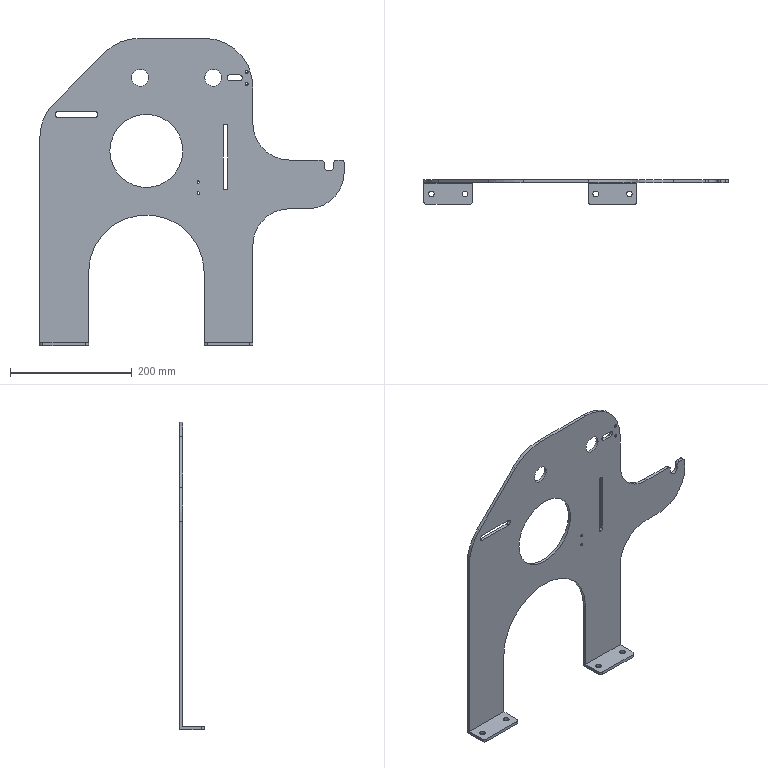Component | SolidWorks | MirrorVerticalPlate_Default_ByProcessing-5 | 1 solid | 76 faces | volume 665650 mm3 | cylinder 45 | plane 27 | cone 4 | commonest cylinder face diameters 10 x13 9.225 x8 120 x5 4 x4 4.2 x4 28 x4 160 x3 8 x2